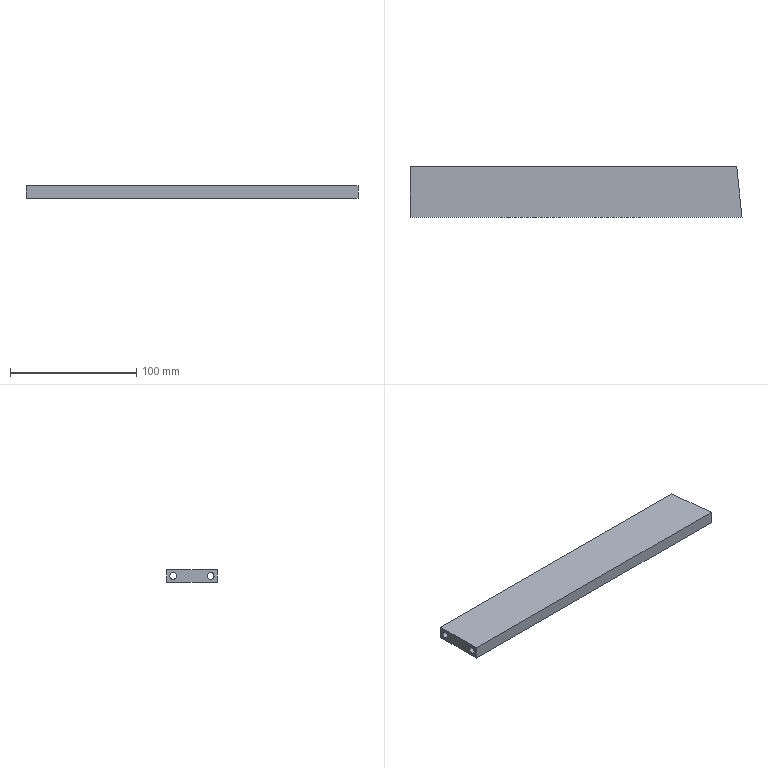CAM job | Mastercam | mm | 6 operations | part box 265.2 x 48.96 x 10
1. Contour (2D) | 9 - 10 平铣刀
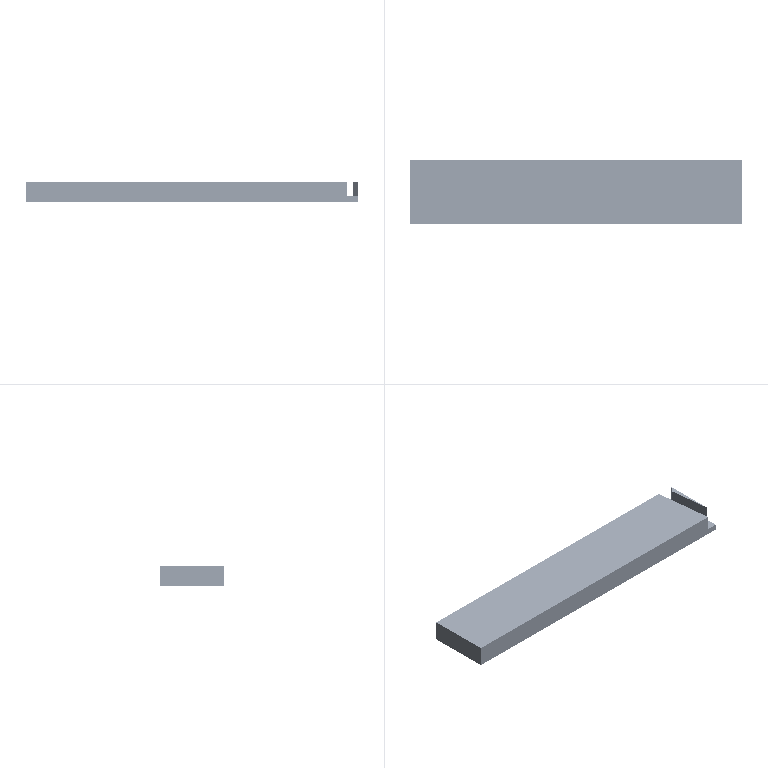2. Contour (2D) | 9 - 10 平铣刀
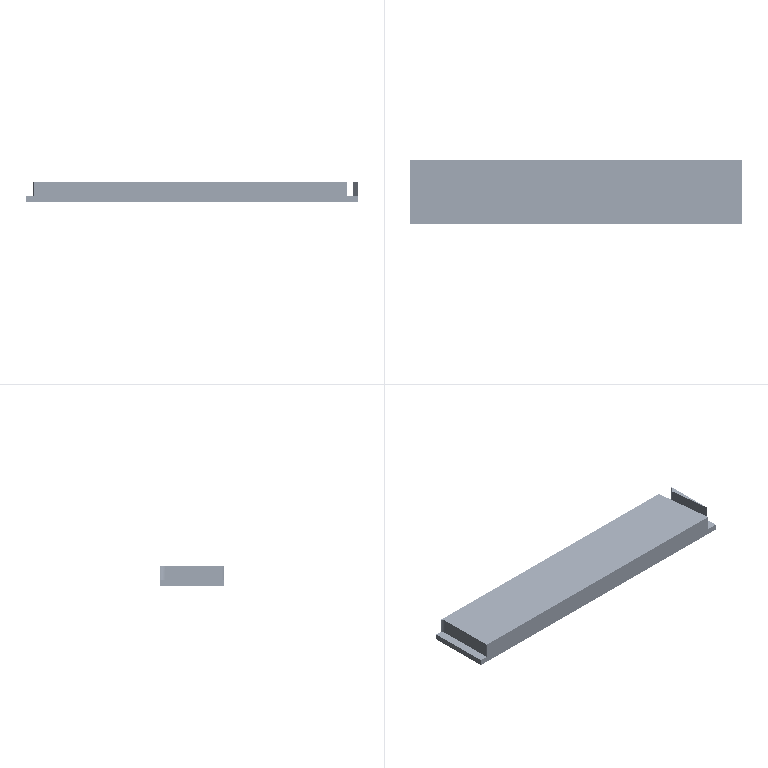3. Drill/Counterbore | 12 - 6 定位钻
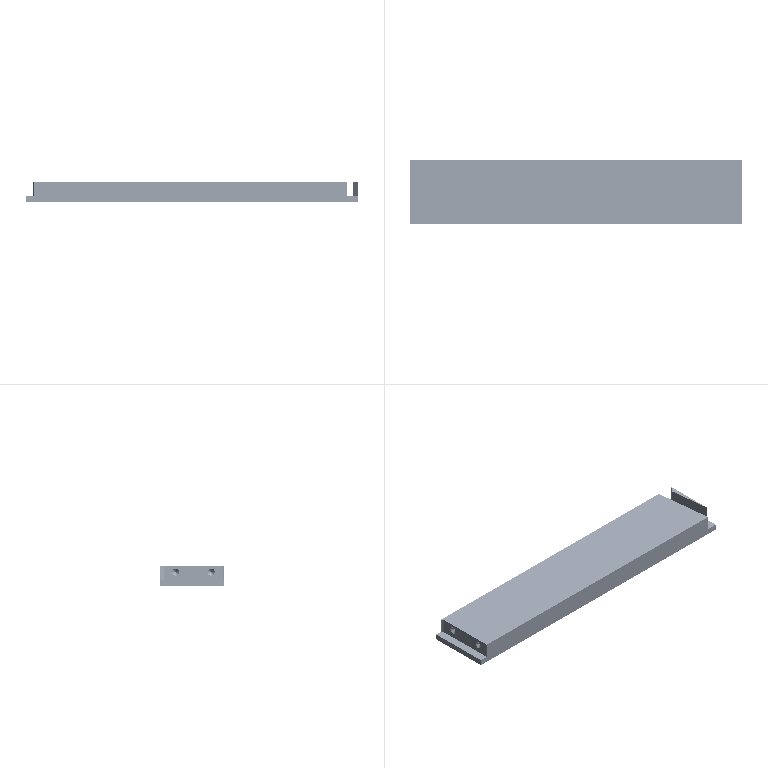4. Peck Drill | 2 - 5.3 钻头
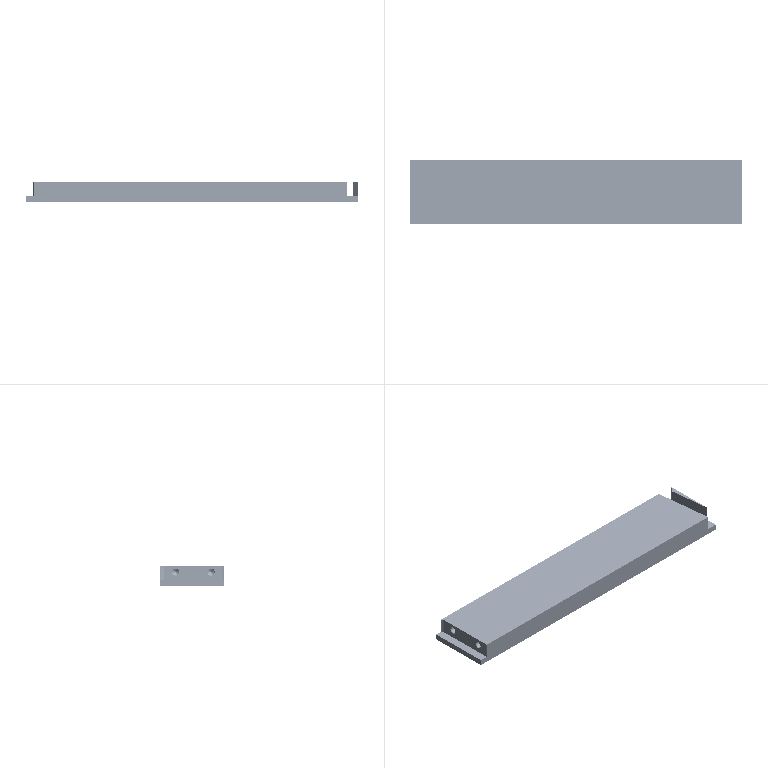5. Drill/Counterbore | 12 - 6 定位钻
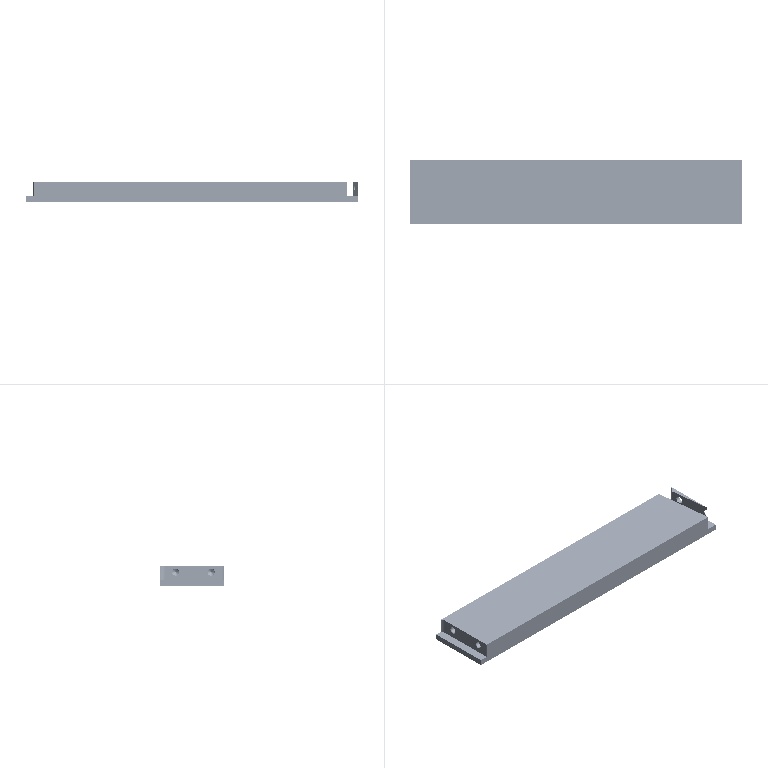6. Peck Drill | 2 - 5.3 钻头